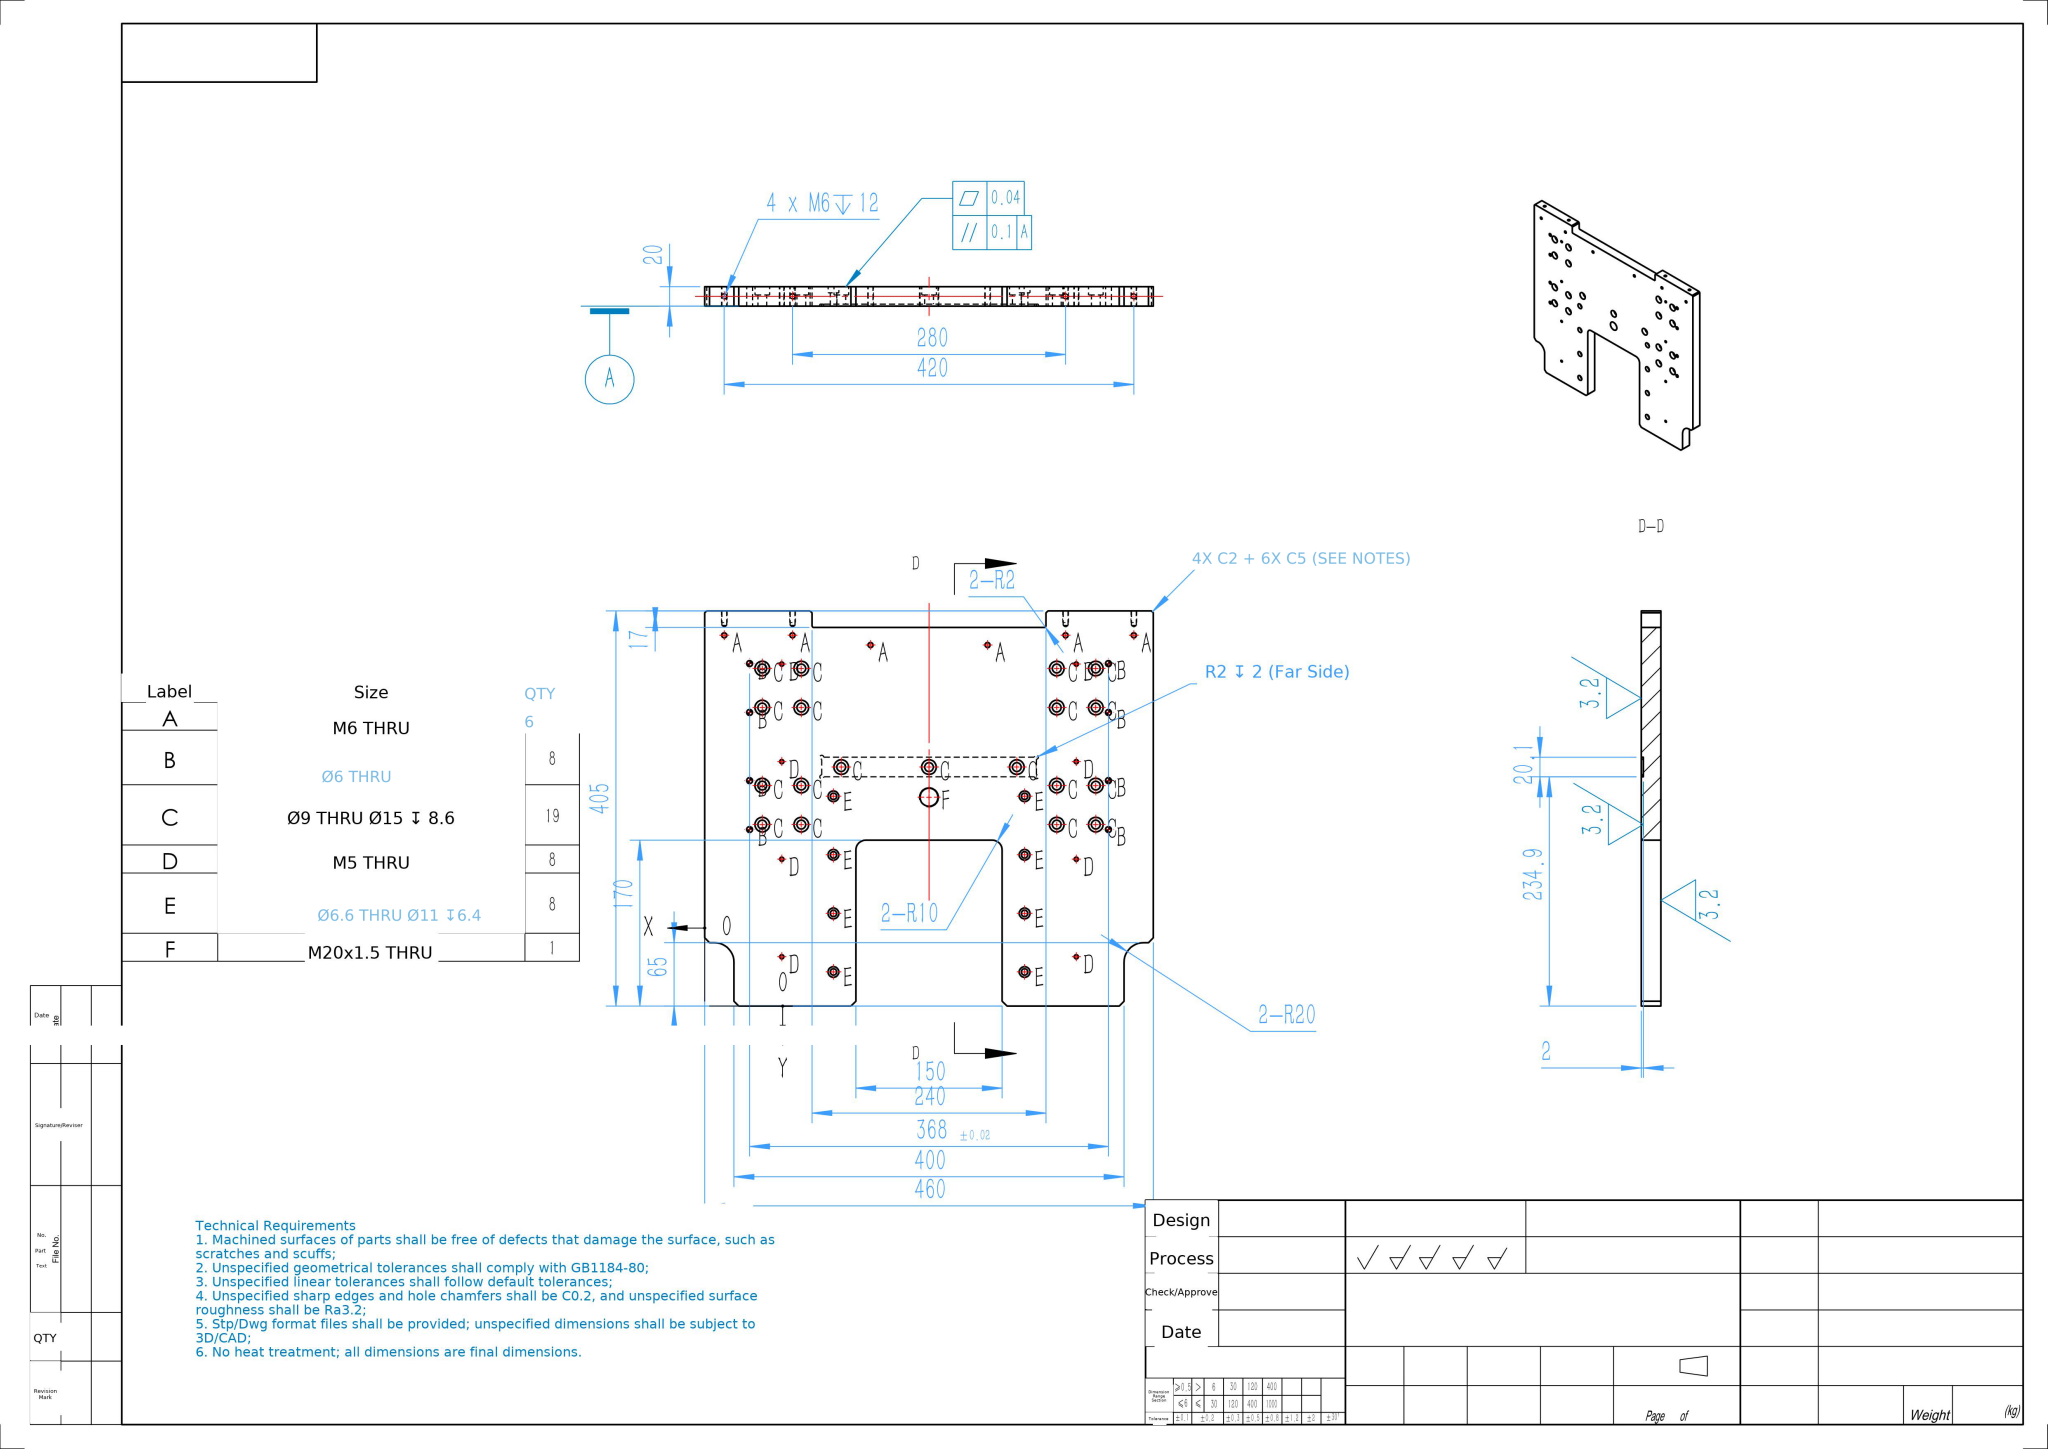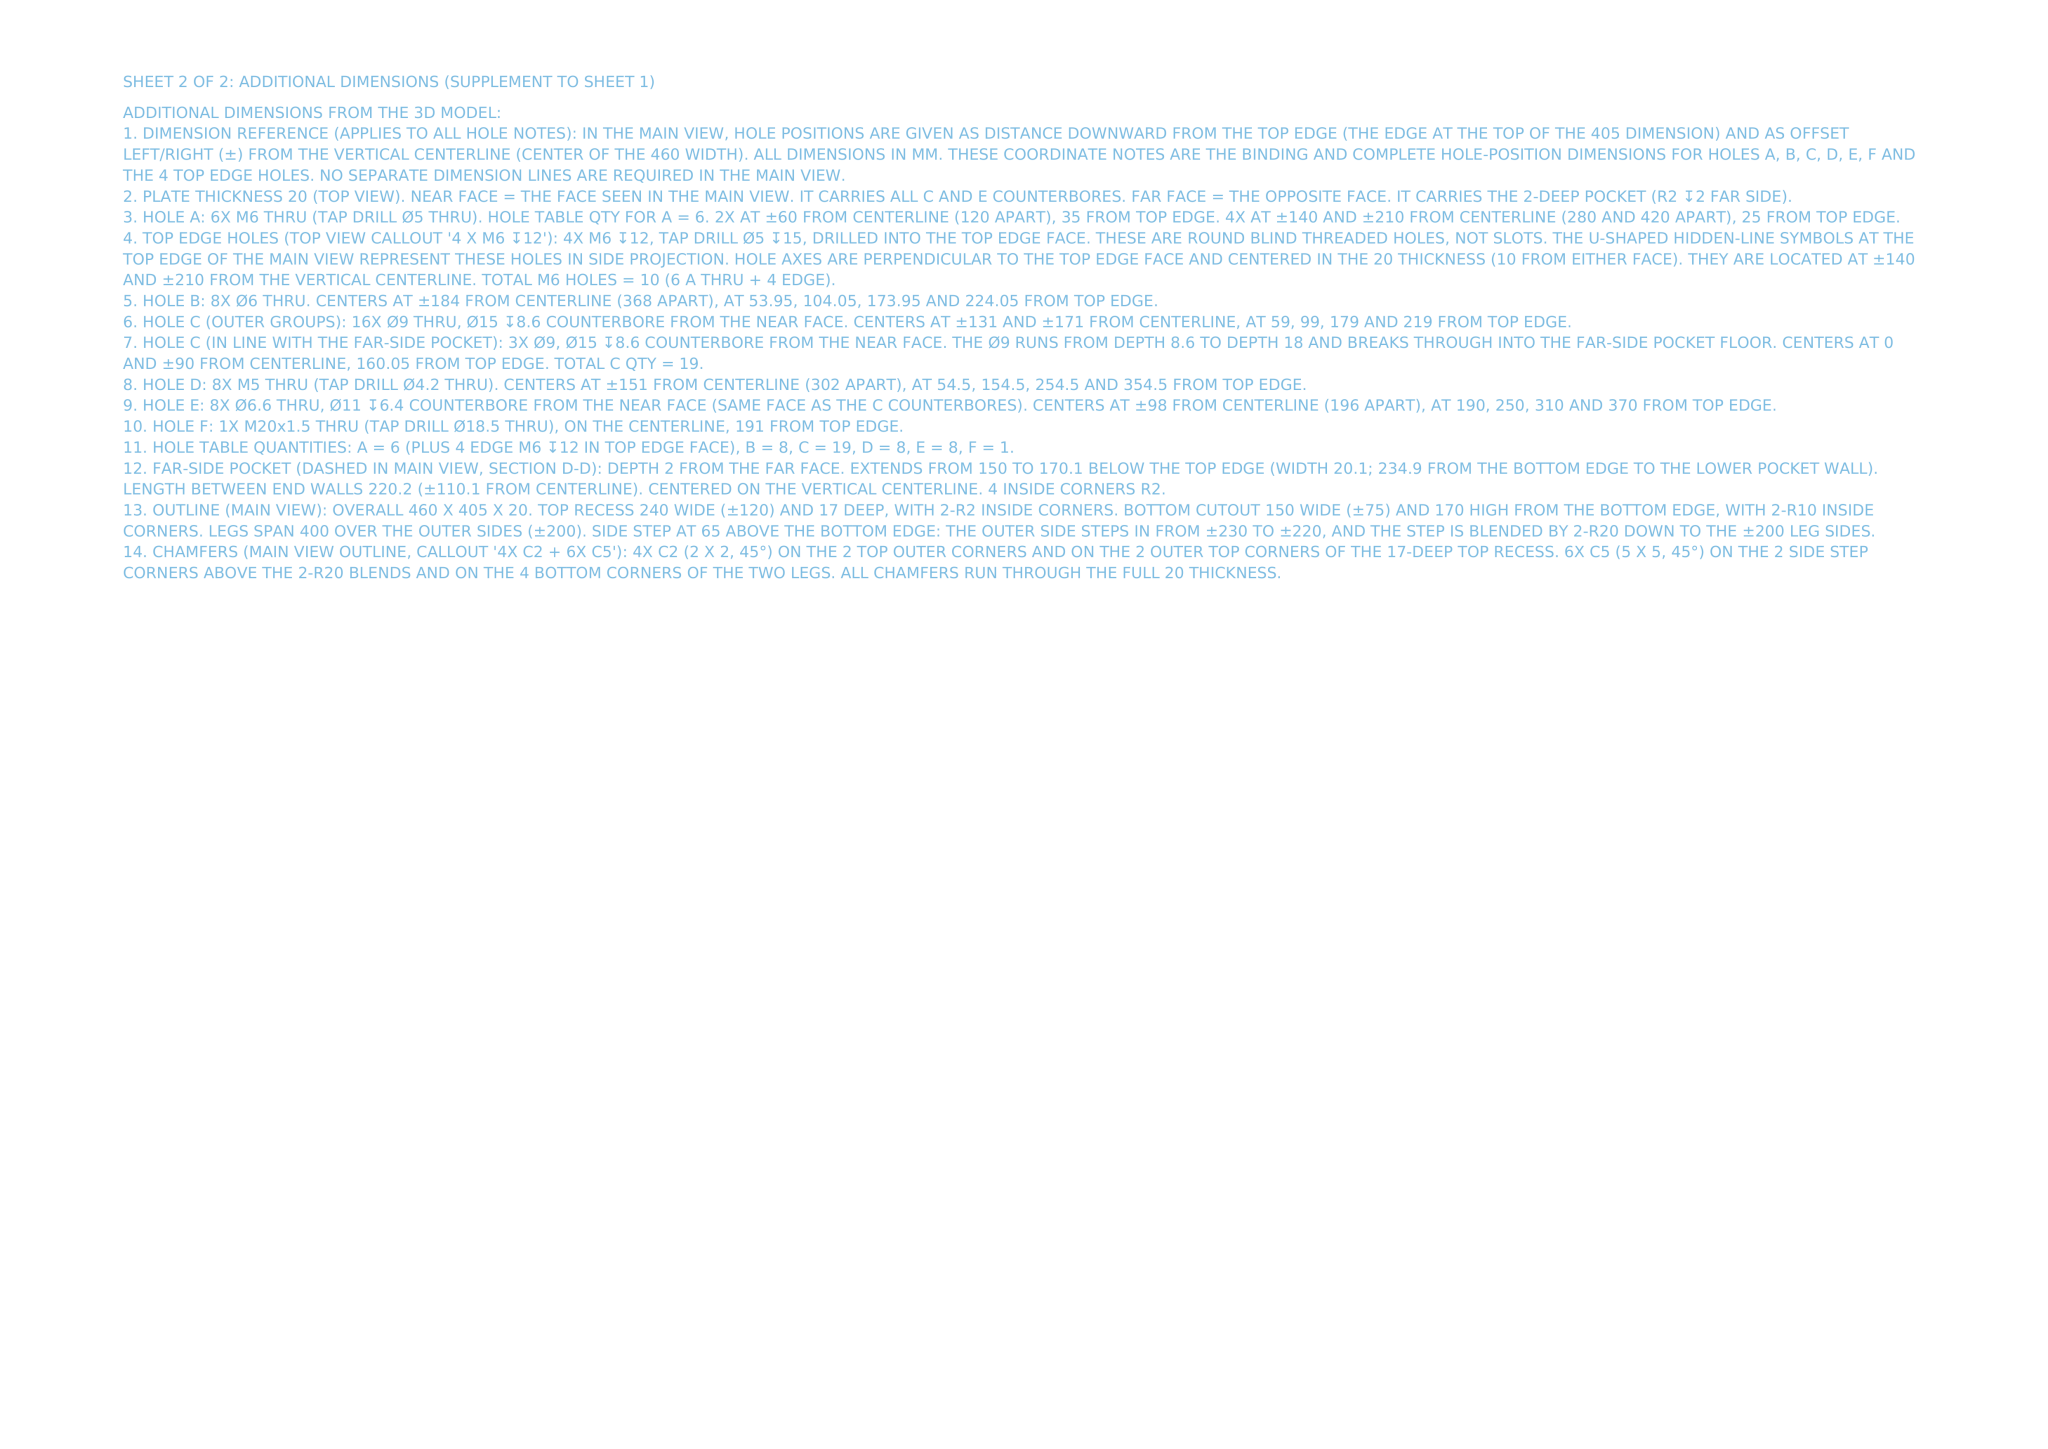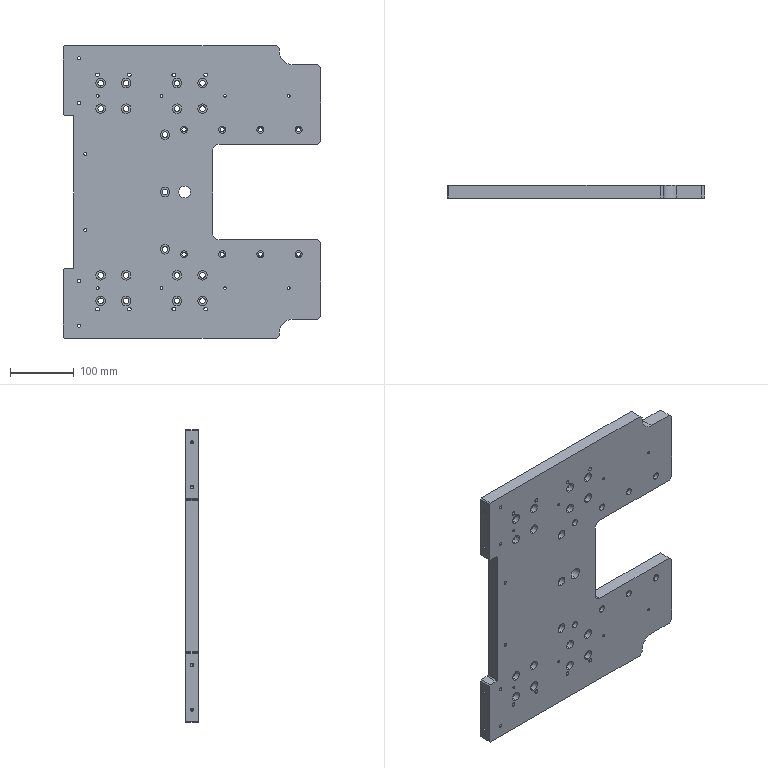Part | NX | mm | 1 solid | 242 faces | box 405 x 20 x 460 mm | volume 2983588 mm3 | cylinder 174 | plane 60 | cone 8 | commonest cylinder face diameters 15 x38 9 x38 5 x20 6 x16 4.2 x16 11 x16 6.6 x16 4 x8